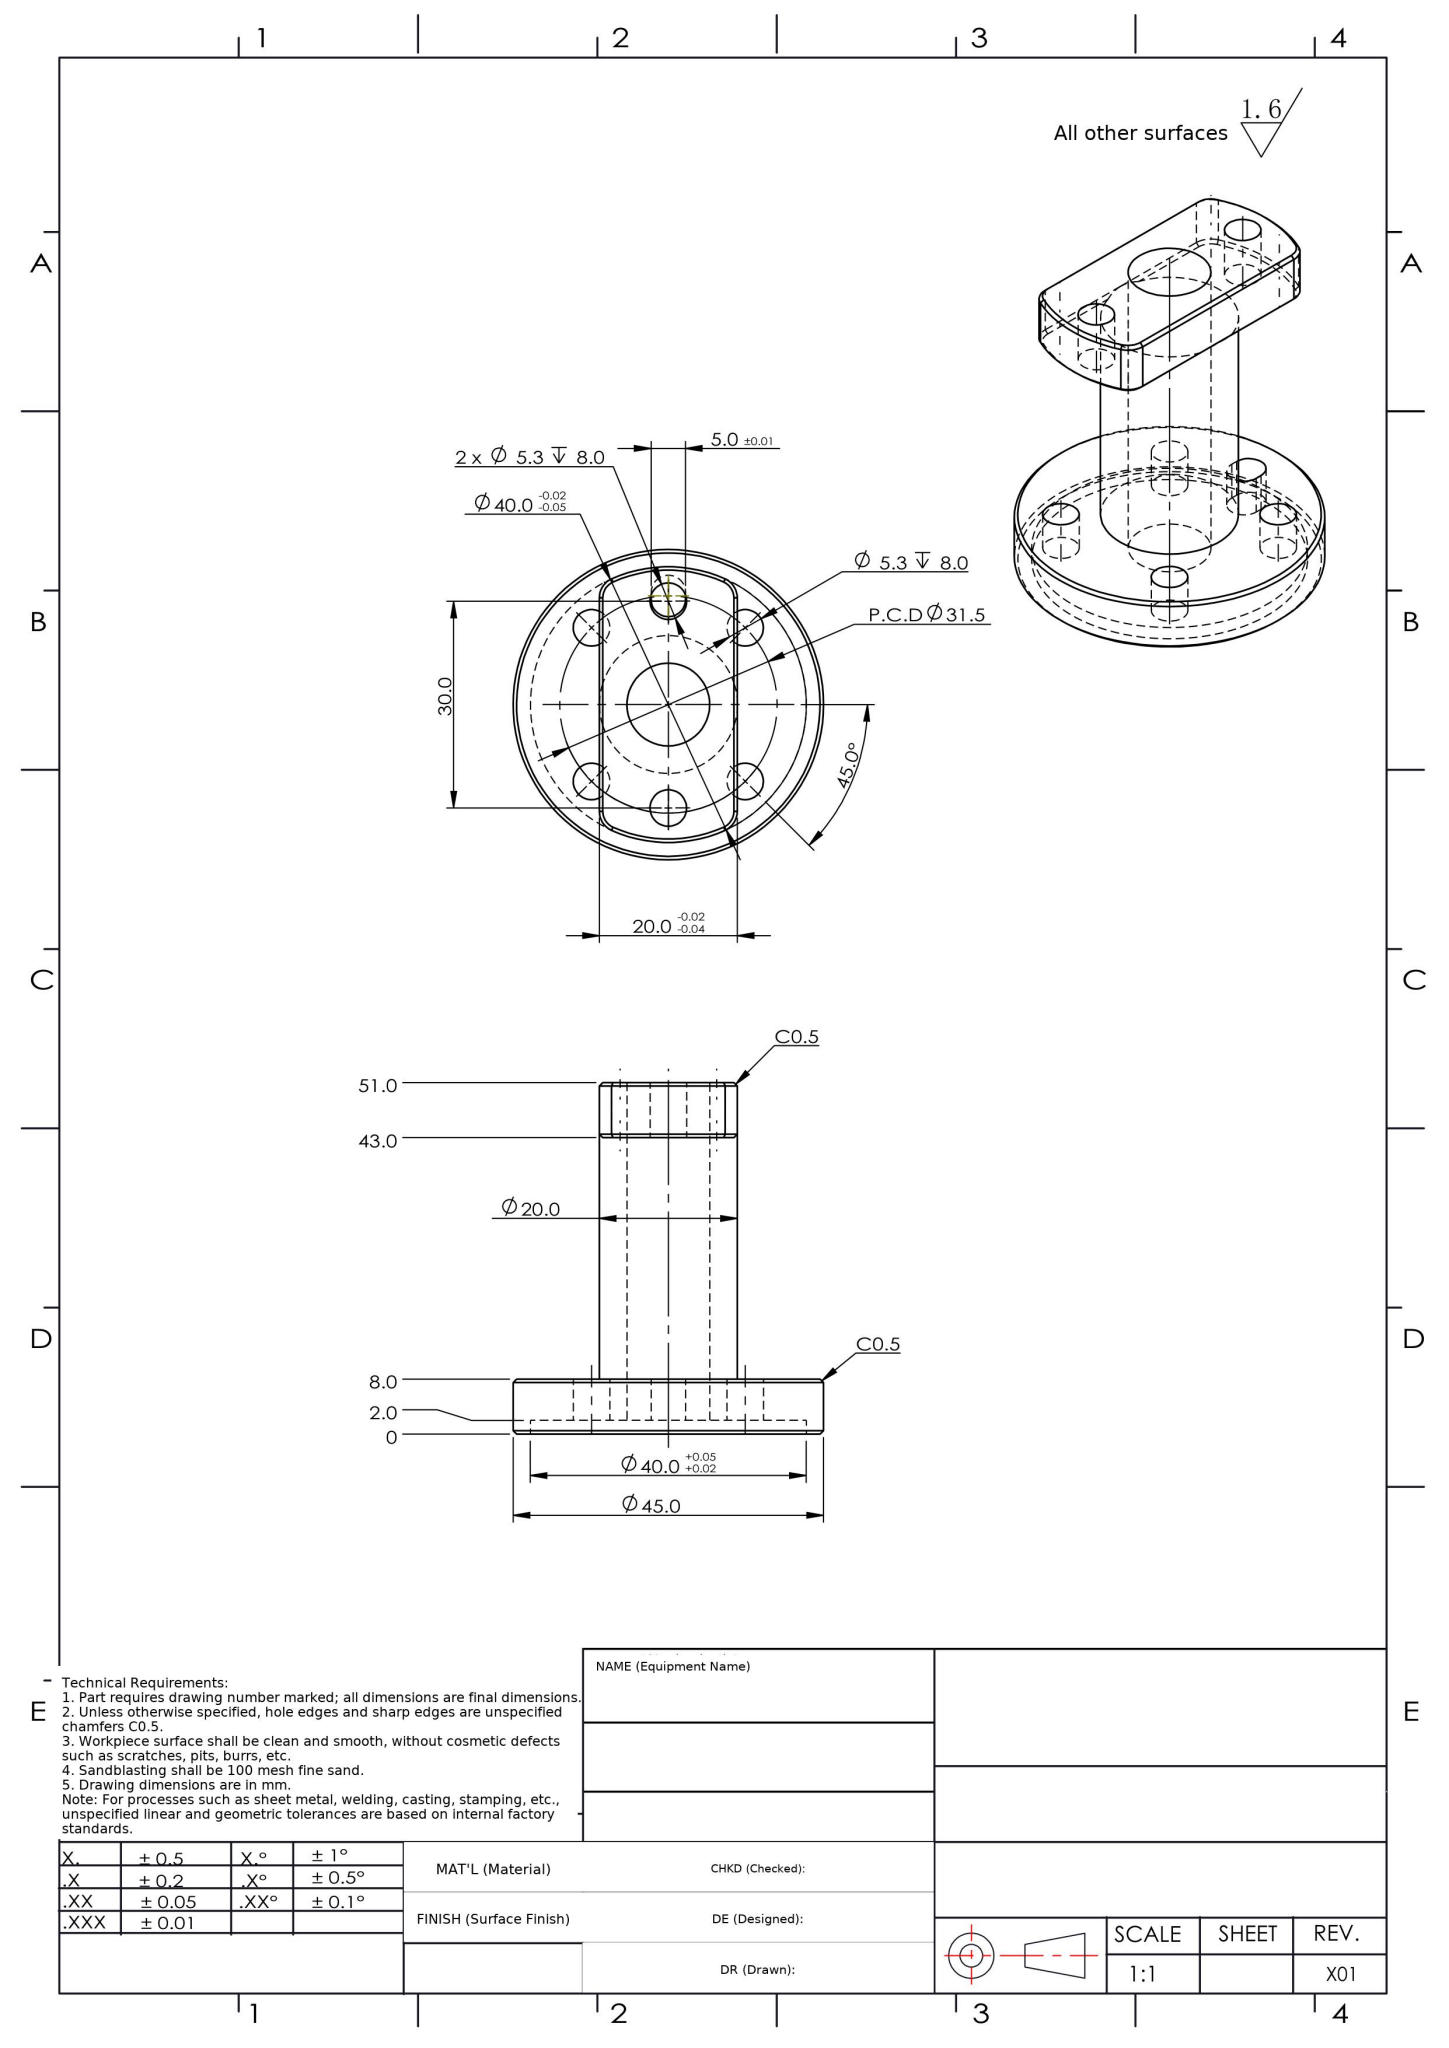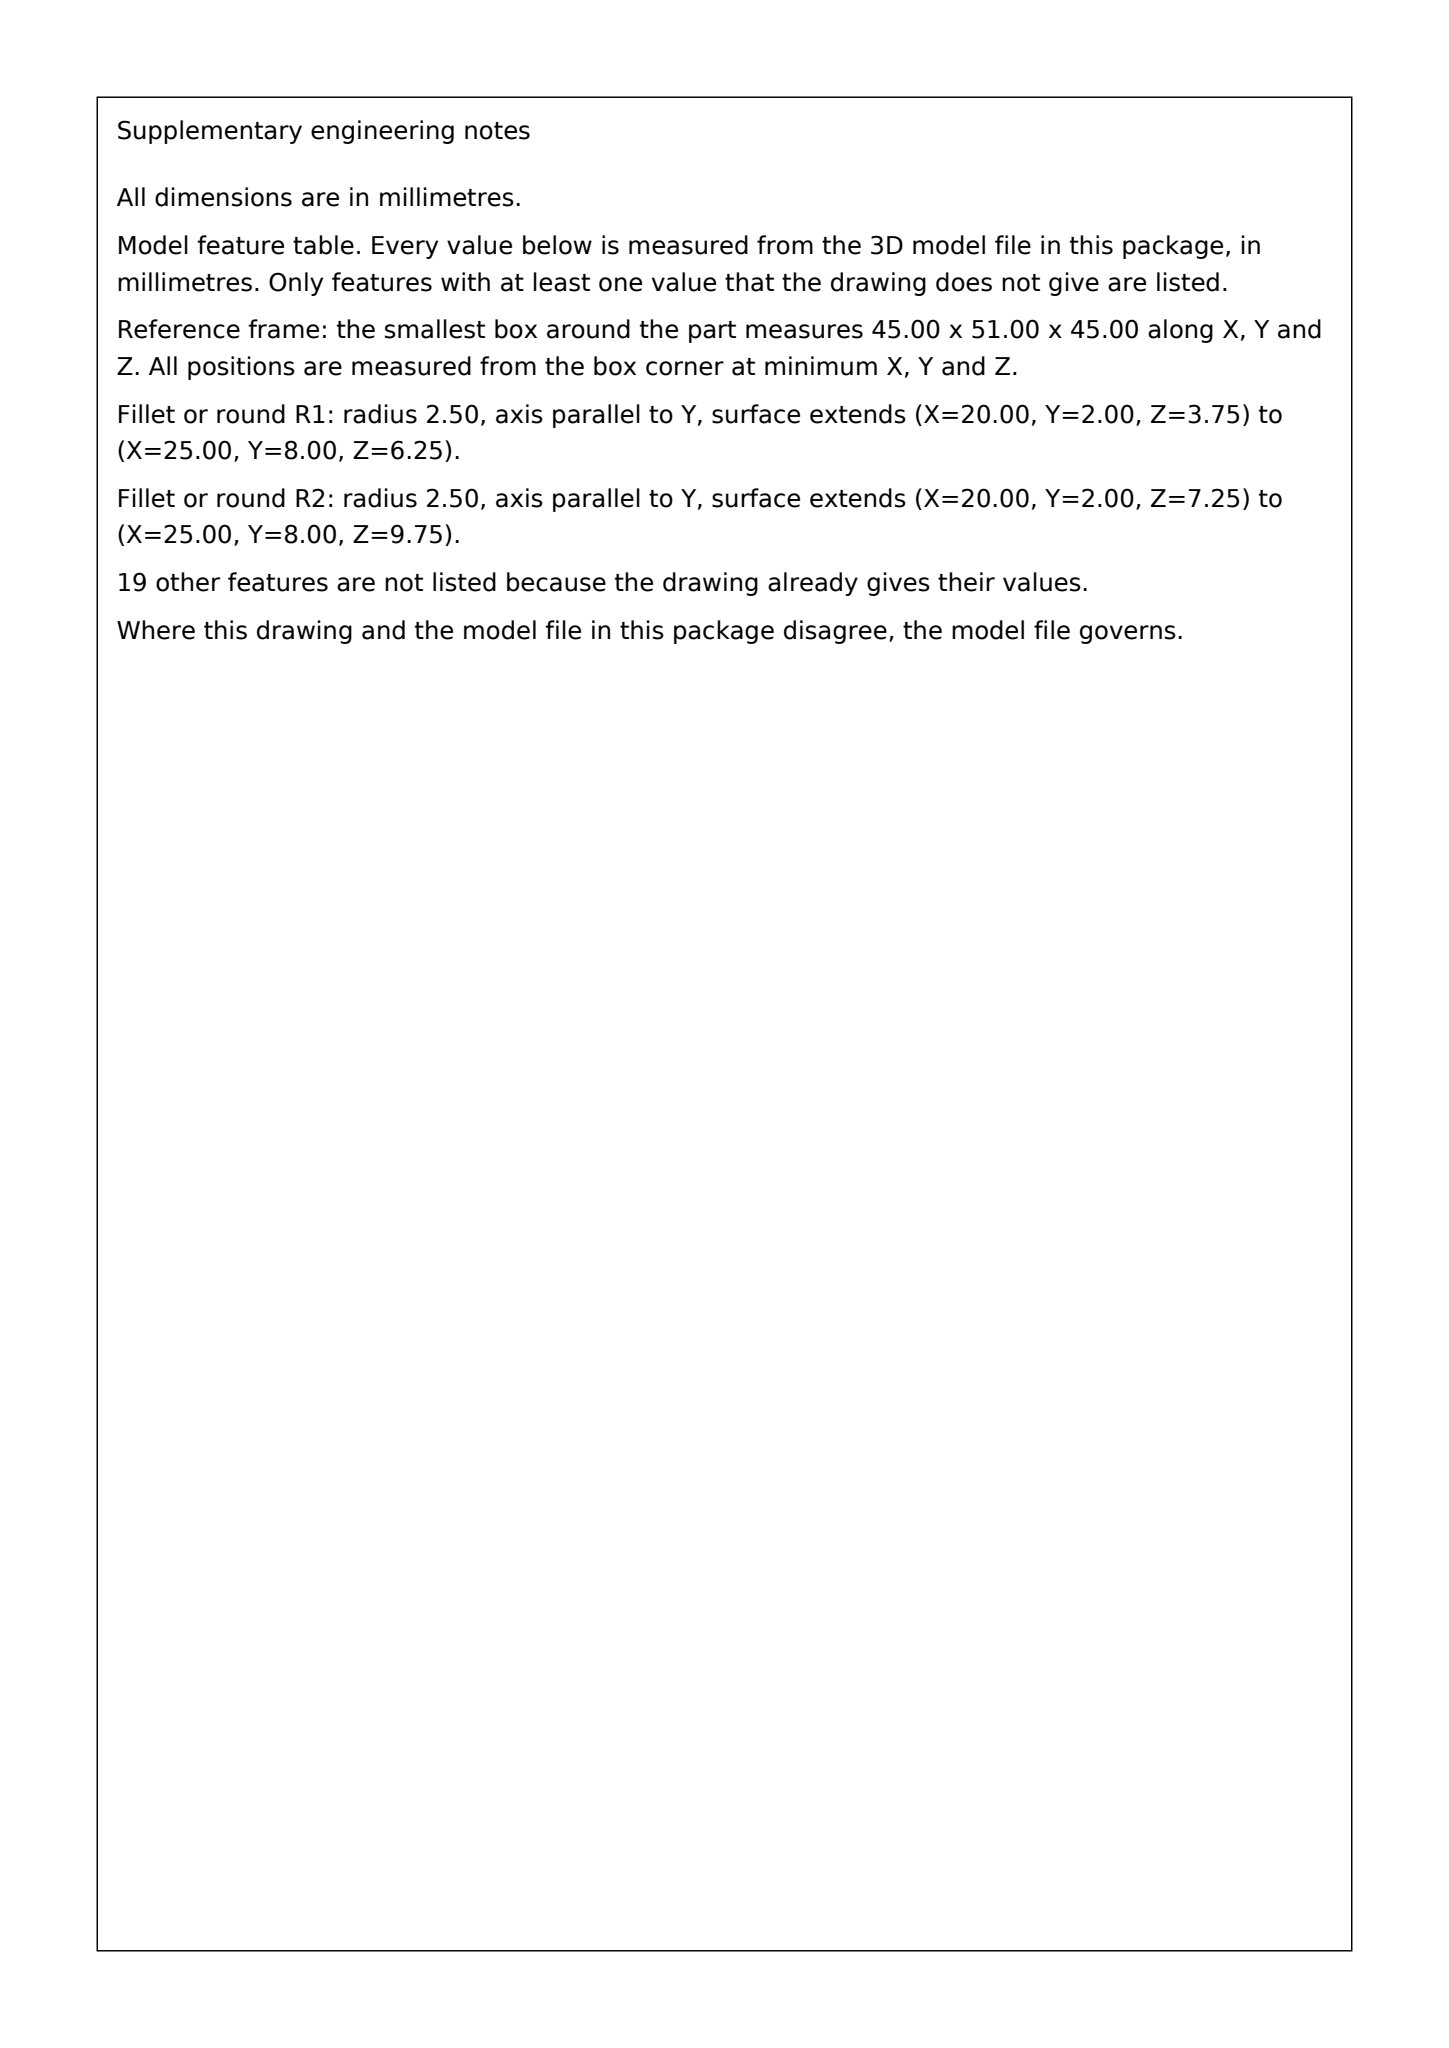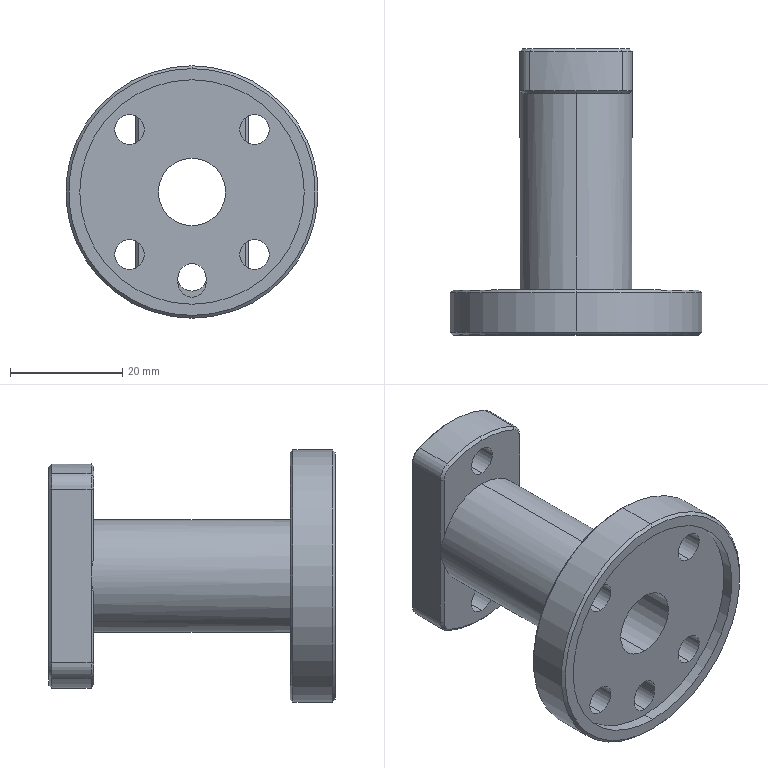Part | SolidWorks | mm | 1 solid | 64 faces | box 45 x 51 x 45 mm | volume 20676 mm3 | cylinder 30 | cone 18 | plane 16 | commonest cylinder face diameters 5.3 x12 40 x5 6 x4 5 x3 20 x2 45 x2 12 x2